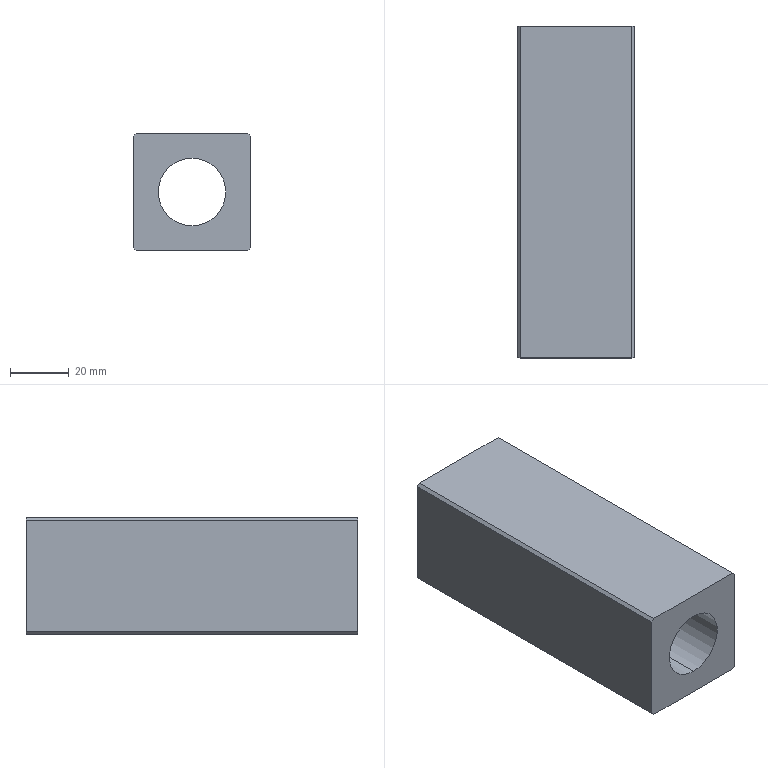Component | SolidWorks | BearingLiftingModule-1_CylinderLiftingModule-1_CDQ2B20-40DZ-L-M9B_0_0_0-1_CHEN123-AA-25-1 | 1 solid | 18 faces | box 40 x 113 x 40 mm | volume 118001 mm3 | plane 12 | cylinder 6 | commonest cylinder face diameters 30 x2 23 x2 28 x2
build123d program:
from build123d import *

# Parameters (mm, degrees)
SKETCH1_W           = 40
SKETCH1_H           = 40
BOSS_EXTRUDE1_DEPTH = 113
SKETCH2_R           = 11.5
CUT_EXTRUDE1_DEPTH  = 117.486
SKETCH3_R           = 14
CUT_EXTRUDE2_DEPTH  = 63
SKETCH4_R           = 15
CUT_EXTRUDE3_DEPTH  = 33
CHAMFER1_SIZE       = 1


with BuildPart() as part:
    # Sketch1 → Boss-Extrude1 (new body)
    with BuildSketch(Plane.XY):
        Rectangle(SKETCH1_W, SKETCH1_H)
    extrude(amount=BOSS_EXTRUDE1_DEPTH)

    # Sketch2 → Cut-Extrude1 (cut, through all)
    with BuildSketch(Plane.XY.offset(113)):
        Circle(SKETCH2_R)
    extrude(amount=-CUT_EXTRUDE1_DEPTH, mode=Mode.SUBTRACT)

    # Sketch3 → Cut-Extrude2 (cut)
    with BuildSketch(Plane(origin=(0, 0, 0), x_dir=(-1, 0, 0), z_dir=(0, 0, -1))):
        Circle(SKETCH3_R)
    extrude(amount=-CUT_EXTRUDE2_DEPTH, mode=Mode.SUBTRACT)

    # Sketch4 → Cut-Extrude3 (cut)
    with BuildSketch(Plane(origin=(0, 0, 0), x_dir=(-1, 0, 0), z_dir=(0, 0, -1))):
        Circle(SKETCH4_R)
    extrude(amount=-CUT_EXTRUDE3_DEPTH, mode=Mode.SUBTRACT)

    # Chamfer1
    chamfer1_edges = [part.edges().sort_by_distance(p)[0] for p in [
        (20, -20, 56.5),
        (-20, -20, 56.5),
        (-20, 20, 56.5),
        (20, 20, 56.5),
    ]]
    chamfer(chamfer1_edges, length=CHAMFER1_SIZE)


solid = part.part

# Placed as in the assembly
solid = solid.moved(Location((69.999, 21.801, 30), (90, 0, 0)))
STEP:
#1=CARTESIAN_POINT('',(2.756,-0.4409,1.772));
#2=VERTEX_POINT('',#1);
#3=CARTESIAN_POINT('',(2.756,-0.4409,0.5906));
#4=VERTEX_POINT('',#3);
#5=CARTESIAN_POINT('',(2.756,-0.4409,1.181));
#6=DIRECTION('',(0.,1.,-0.));
#7=DIRECTION('',(0.,0.,-1.));
#8=AXIS2_PLACEMENT_3D('',#5,#6,#7);
#9=CIRCLE('',#8,0.5906);
#10=EDGE_CURVE('',#2,#4,#9,.T.);
#11=ORIENTED_EDGE('',*,*,#10,.F.);
#12=CARTESIAN_POINT('',(2.756,0.8583,1.772));
#13=VERTEX_POINT('',#12);
#14=CARTESIAN_POINT('',(2.756,-0.4409,1.772));
#15=DIRECTION('',(0.,1.,-0.));
#16=VECTOR('',#15,39.37);
#17=LINE('',#14,#16);
#18=EDGE_CURVE('',#2,#13,#17,.T.);
#19=ORIENTED_EDGE('',*,*,#18,.T.);
#20=CARTESIAN_POINT('',(2.756,0.8583,0.5906));
#21=VERTEX_POINT('',#20);
#22=CARTESIAN_POINT('',(2.756,0.8583,1.181));
#23=DIRECTION('',(0.,1.,-0.));
#24=DIRECTION('',(0.,0.,-1.));
#25=AXIS2_PLACEMENT_3D('',#22,#23,#24);
#26=CIRCLE('',#25,0.5906);
#27=EDGE_CURVE('',#13,#21,#26,.T.);
#28=ORIENTED_EDGE('',*,*,#27,.T.);
#29=CARTESIAN_POINT('',(2.756,-0.4409,0.5906));
#30=DIRECTION('',(0.,1.,-0.));
#31=VECTOR('',#30,39.37);
#32=LINE('',#29,#31);
#33=EDGE_CURVE('',#4,#21,#32,.T.);
#34=ORIENTED_EDGE('',*,*,#33,.F.);
#35=EDGE_LOOP('',(#11,#19,#28,#34));
#36=FACE_OUTER_BOUND('',#35,.T.);
#37=CARTESIAN_POINT('',(2.756,-0.4409,1.181));
#38=DIRECTION('',(0.,1.,-0.));
#39=DIRECTION('',(0.,0.,-1.));
#40=AXIS2_PLACEMENT_3D('',#37,#38,#39);
#41=CYLINDRICAL_SURFACE('',#40,0.5906);
#42=ADVANCED_FACE('',(#36),#41,.F.);
#43=CARTESIAN_POINT('',(2.756,-1.622,0.7283));
#44=VERTEX_POINT('',#43);
#45=CARTESIAN_POINT('',(2.756,-1.622,1.634));
#46=VERTEX_POINT('',#45);
#47=CARTESIAN_POINT('',(2.756,-1.622,1.181));
#48=DIRECTION('',(0.,-1.,0.));
#49=DIRECTION('',(0.,0.,-1.));
#50=AXIS2_PLACEMENT_3D('',#47,#48,#49);
#51=CIRCLE('',#50,0.4528);
#52=EDGE_CURVE('',#44,#46,#51,.T.);
#53=ORIENTED_EDGE('',*,*,#52,.F.);
#54=CARTESIAN_POINT('',(2.756,-3.591,0.7283));
#55=VERTEX_POINT('',#54);
#56=CARTESIAN_POINT('',(2.756,0.8583,0.7283));
#57=DIRECTION('',(0.,-1.,0.));
#58=VECTOR('',#57,39.37);
#59=LINE('',#56,#58);
#60=EDGE_CURVE('',#44,#55,#59,.T.);
#61=ORIENTED_EDGE('',*,*,#60,.T.);
#62=CARTESIAN_POINT('',(2.756,-3.591,1.634));
#63=VERTEX_POINT('',#62);
#64=CARTESIAN_POINT('',(2.756,-3.591,1.181));
#65=DIRECTION('',(0.,-1.,0.));
#66=DIRECTION('',(0.,0.,1.));
#67=AXIS2_PLACEMENT_3D('',#64,#65,#66);
#68=CIRCLE('',#67,0.4528);
#69=EDGE_CURVE('',#55,#63,#68,.T.);
#70=ORIENTED_EDGE('',*,*,#69,.T.);
#71=CARTESIAN_POINT('',(2.756,0.8583,1.634));
#72=DIRECTION('',(0.,-1.,0.));
#73=VECTOR('',#72,39.37);
#74=LINE('',#71,#73);
#75=EDGE_CURVE('',#46,#63,#74,.T.);
#76=ORIENTED_EDGE('',*,*,#75,.F.);
#77=EDGE_LOOP('',(#53,#61,#70,#76));
#78=FACE_OUTER_BOUND('',#77,.T.);
#79=CARTESIAN_POINT('',(2.756,0.8583,1.181));
#80=DIRECTION('',(0.,-1.,0.));
#81=DIRECTION('',(0.,0.,1.));
#82=AXIS2_PLACEMENT_3D('',#79,#80,#81);
#83=CYLINDRICAL_SURFACE('',#82,0.4528);
#84=ADVANCED_FACE('',(#78),#83,.F.);
#85=CARTESIAN_POINT('',(2.756,-1.622,1.732));
#86=VERTEX_POINT('',#85);
#87=CARTESIAN_POINT('',(2.756,-1.622,0.6299));
#88=VERTEX_POINT('',#87);
#89=CARTESIAN_POINT('',(2.756,-1.622,1.181));
#90=DIRECTION('',(0.,1.,-0.));
#91=DIRECTION('',(0.,0.,-1.));
#92=AXIS2_PLACEMENT_3D('',#89,#90,#91);
#93=CIRCLE('',#92,0.5512);
#94=EDGE_CURVE('',#86,#88,#93,.T.);
#95=ORIENTED_EDGE('',*,*,#94,.F.);
#96=CARTESIAN_POINT('',(2.756,-0.4409,1.732));
#97=VERTEX_POINT('',#96);
#98=CARTESIAN_POINT('',(2.756,-1.622,1.732));
#99=DIRECTION('',(0.,1.,-0.));
#100=VECTOR('',#99,39.37);
#101=LINE('',#98,#100);
#102=EDGE_CURVE('',#86,#97,#101,.T.);
#103=ORIENTED_EDGE('',*,*,#102,.T.);
#104=CARTESIAN_POINT('',(2.756,-0.4409,0.6299));
#105=VERTEX_POINT('',#104);
#106=CARTESIAN_POINT('',(2.756,-0.4409,1.181));
#107=DIRECTION('',(0.,-1.,0.));
#108=DIRECTION('',(0.,0.,-1.));
#109=AXIS2_PLACEMENT_3D('',#106,#107,#108);
#110=CIRCLE('',#109,0.5512);
#111=EDGE_CURVE('',#105,#97,#110,.T.);
#112=ORIENTED_EDGE('',*,*,#111,.F.);
#113=CARTESIAN_POINT('',(2.756,-1.622,0.6299));
#114=DIRECTION('',(0.,1.,-0.));
#115=VECTOR('',#114,39.37);
#116=LINE('',#113,#115);
#117=EDGE_CURVE('',#88,#105,#116,.T.);
#118=ORIENTED_EDGE('',*,*,#117,.F.);
#119=EDGE_LOOP('',(#95,#103,#112,#118));
#120=FACE_OUTER_BOUND('',#119,.T.);
#121=CARTESIAN_POINT('',(2.756,-1.622,1.181));
#122=DIRECTION('',(0.,1.,-0.));
#123=DIRECTION('',(0.,0.,-1.));
#124=AXIS2_PLACEMENT_3D('',#121,#122,#123);
#125=CYLINDRICAL_SURFACE('',#124,0.5512);
#126=ADVANCED_FACE('',(#120),#125,.F.);
#127=ORIENTED_EDGE('',*,*,#102,.F.);
#128=CARTESIAN_POINT('',(2.756,-1.622,1.181));
#129=DIRECTION('',(0.,1.,-0.));
#130=DIRECTION('',(0.,0.,-1.));
#131=AXIS2_PLACEMENT_3D('',#128,#129,#130);
#132=CIRCLE('',#131,0.5512);
#133=EDGE_CURVE('',#88,#86,#132,.T.);
#134=ORIENTED_EDGE('',*,*,#133,.F.);
#135=ORIENTED_EDGE('',*,*,#117,.T.);
#136=CARTESIAN_POINT('',(2.756,-0.4409,1.181));
#137=DIRECTION('',(0.,-1.,0.));
#138=DIRECTION('',(0.,0.,-1.));
#139=AXIS2_PLACEMENT_3D('',#136,#137,#138);
#140=CIRCLE('',#139,0.5512);
#141=EDGE_CURVE('',#97,#105,#140,.T.);
#142=ORIENTED_EDGE('',*,*,#141,.F.);
#143=EDGE_LOOP('',(#127,#134,#135,#142));
#144=FACE_OUTER_BOUND('',#143,.T.);
#145=CARTESIAN_POINT('',(2.756,-1.622,1.181));
#146=DIRECTION('',(0.,1.,-0.));
#147=DIRECTION('',(0.,0.,-1.));
#148=AXIS2_PLACEMENT_3D('',#145,#146,#147);
#149=CYLINDRICAL_SURFACE('',#148,0.5512);
#150=ADVANCED_FACE('',(#144),#149,.F.);
#151=ORIENTED_EDGE('',*,*,#60,.F.);
#152=CARTESIAN_POINT('',(2.756,-1.622,1.181));
#153=DIRECTION('',(0.,-1.,0.));
#154=DIRECTION('',(0.,0.,-1.));
#155=AXIS2_PLACEMENT_3D('',#152,#153,#154);
#156=CIRCLE('',#155,0.4528);
#157=EDGE_CURVE('',#46,#44,#156,.T.);
#158=ORIENTED_EDGE('',*,*,#157,.F.);
#159=ORIENTED_EDGE('',*,*,#75,.T.);
#160=CARTESIAN_POINT('',(2.756,-3.591,1.181));
#161=DIRECTION('',(0.,-1.,0.));
#162=DIRECTION('',(0.,0.,1.));
#163=AXIS2_PLACEMENT_3D('',#160,#161,#162);
#164=CIRCLE('',#163,0.4528);
#165=EDGE_CURVE('',#63,#55,#164,.T.);
#166=ORIENTED_EDGE('',*,*,#165,.T.);
#167=EDGE_LOOP('',(#151,#158,#159,#166));
#168=FACE_OUTER_BOUND('',#167,.T.);
#169=CARTESIAN_POINT('',(2.756,0.8583,1.181));
#170=DIRECTION('',(0.,-1.,0.));
#171=DIRECTION('',(0.,0.,1.));
#172=AXIS2_PLACEMENT_3D('',#169,#170,#171);
#173=CYLINDRICAL_SURFACE('',#172,0.4528);
#174=ADVANCED_FACE('',(#168),#173,.F.);
#175=CARTESIAN_POINT('',(3.504,0.8583,1.969));
#176=VERTEX_POINT('',#175);
#177=CARTESIAN_POINT('',(2.008,0.8583,1.969));
#178=VERTEX_POINT('',#177);
#179=CARTESIAN_POINT('',(3.543,0.8583,1.969));
#180=DIRECTION('',(-1.,0.,0.));
#181=VECTOR('',#180,39.37);
#182=LINE('',#179,#181);
#183=EDGE_CURVE('',#176,#178,#182,.T.);
#184=ORIENTED_EDGE('',*,*,#183,.T.);
#185=CARTESIAN_POINT('',(2.008,-3.591,1.969));
#186=VERTEX_POINT('',#185);
#187=CARTESIAN_POINT('',(2.008,-3.591,1.969));
#188=DIRECTION('',(0.,-1.,0.));
#189=VECTOR('',#188,39.37);
#190=LINE('',#187,#189);
#191=EDGE_CURVE('',#178,#186,#190,.T.);
#192=ORIENTED_EDGE('',*,*,#191,.T.);
#193=CARTESIAN_POINT('',(3.504,-3.591,1.969));
#194=VERTEX_POINT('',#193);
#195=CARTESIAN_POINT('',(3.543,-3.591,1.969));
#196=DIRECTION('',(-1.,0.,0.));
#197=VECTOR('',#196,39.37);
#198=LINE('',#195,#197);
#199=EDGE_CURVE('',#194,#186,#198,.T.);
#200=ORIENTED_EDGE('',*,*,#199,.F.);
#201=CARTESIAN_POINT('',(3.504,-3.591,1.969));
#202=DIRECTION('',(0.,1.,-0.));
#203=VECTOR('',#202,39.37);
#204=LINE('',#201,#203);
#205=EDGE_CURVE('',#194,#176,#204,.T.);
#206=ORIENTED_EDGE('',*,*,#205,.T.);
#207=EDGE_LOOP('',(#184,#192,#200,#206));
#208=FACE_OUTER_BOUND('',#207,.T.);
#209=CARTESIAN_POINT('',(3.543,-3.591,1.969));
#210=DIRECTION('',(-0.,-0.,-1.));
#211=DIRECTION('',(0.,-1.,0.));
#212=AXIS2_PLACEMENT_3D('',#209,#210,#211);
#213=PLANE('',#212);
#214=ADVANCED_FACE('',(#208),#213,.F.);
#215=CARTESIAN_POINT('',(1.968,0.8583,1.929));
#216=VERTEX_POINT('',#215);
#217=CARTESIAN_POINT('',(1.968,0.8583,0.4331));
#218=VERTEX_POINT('',#217);
#219=CARTESIAN_POINT('',(1.968,0.8583,0.3937));
#220=DIRECTION('',(-0.,-0.,-1.));
#221=VECTOR('',#220,39.37);
#222=LINE('',#219,#221);
#223=EDGE_CURVE('',#216,#218,#222,.T.);
#224=ORIENTED_EDGE('',*,*,#223,.T.);
#225=CARTESIAN_POINT('',(1.968,-3.591,0.4331));
#226=VERTEX_POINT('',#225);
#227=CARTESIAN_POINT('',(1.968,-3.591,0.4331));
#228=DIRECTION('',(0.,-1.,0.));
#229=VECTOR('',#228,39.37);
#230=LINE('',#227,#229);
#231=EDGE_CURVE('',#218,#226,#230,.T.);
#232=ORIENTED_EDGE('',*,*,#231,.T.);
#233=CARTESIAN_POINT('',(1.968,-3.591,1.929));
#234=VERTEX_POINT('',#233);
#235=CARTESIAN_POINT('',(1.968,-3.591,0.3937));
#236=DIRECTION('',(-0.,-0.,-1.));
#237=VECTOR('',#236,39.37);
#238=LINE('',#235,#237);
#239=EDGE_CURVE('',#234,#226,#238,.T.);
#240=ORIENTED_EDGE('',*,*,#239,.F.);
#241=CARTESIAN_POINT('',(1.968,-3.591,1.929));
#242=DIRECTION('',(0.,1.,-0.));
#243=VECTOR('',#242,39.37);
#244=LINE('',#241,#243);
#245=EDGE_CURVE('',#234,#216,#244,.T.);
#246=ORIENTED_EDGE('',*,*,#245,.T.);
#247=EDGE_LOOP('',(#224,#232,#240,#246));
#248=FACE_OUTER_BOUND('',#247,.T.);
#249=CARTESIAN_POINT('',(1.968,-3.591,0.3937));
#250=DIRECTION('',(1.,-0.,-0.));
#251=DIRECTION('',(0.,1.,-0.));
#252=AXIS2_PLACEMENT_3D('',#249,#250,#251);
#253=PLANE('',#252);
#254=ADVANCED_FACE('',(#248),#253,.F.);
#255=CARTESIAN_POINT('',(2.008,0.8583,0.3937));
#256=VERTEX_POINT('',#255);
#257=CARTESIAN_POINT('',(3.504,0.8583,0.3937));
#258=VERTEX_POINT('',#257);
#259=CARTESIAN_POINT('',(3.543,0.8583,0.3937));
#260=DIRECTION('',(1.,0.,-0.));
#261=VECTOR('',#260,39.37);
#262=LINE('',#259,#261);
#263=EDGE_CURVE('',#256,#258,#262,.T.);
#264=ORIENTED_EDGE('',*,*,#263,.T.);
#265=CARTESIAN_POINT('',(3.504,-3.591,0.3937));
#266=VERTEX_POINT('',#265);
#267=CARTESIAN_POINT('',(3.504,-3.591,0.3937));
#268=DIRECTION('',(0.,-1.,0.));
#269=VECTOR('',#268,39.37);
#270=LINE('',#267,#269);
#271=EDGE_CURVE('',#258,#266,#270,.T.);
#272=ORIENTED_EDGE('',*,*,#271,.T.);
#273=CARTESIAN_POINT('',(2.008,-3.591,0.3937));
#274=VERTEX_POINT('',#273);
#275=CARTESIAN_POINT('',(3.543,-3.591,0.3937));
#276=DIRECTION('',(1.,0.,-0.));
#277=VECTOR('',#276,39.37);
#278=LINE('',#275,#277);
#279=EDGE_CURVE('',#274,#266,#278,.T.);
#280=ORIENTED_EDGE('',*,*,#279,.F.);
#281=CARTESIAN_POINT('',(2.008,-3.591,0.3937));
#282=DIRECTION('',(0.,1.,-0.));
#283=VECTOR('',#282,39.37);
#284=LINE('',#281,#283);
#285=EDGE_CURVE('',#274,#256,#284,.T.);
#286=ORIENTED_EDGE('',*,*,#285,.T.);
#287=EDGE_LOOP('',(#264,#272,#280,#286));
#288=FACE_OUTER_BOUND('',#287,.T.);
#289=CARTESIAN_POINT('',(3.543,-3.591,0.3937));
#290=DIRECTION('',(0.,0.,1.));
#291=DIRECTION('',(0.,1.,-0.));
#292=AXIS2_PLACEMENT_3D('',#289,#290,#291);
#293=PLANE('',#292);
#294=ADVANCED_FACE('',(#288),#293,.F.);
#295=CARTESIAN_POINT('',(3.543,-3.591,0.4331));
#296=VERTEX_POINT('',#295);
#297=CARTESIAN_POINT('',(3.543,-3.591,1.929));
#298=VERTEX_POINT('',#297);
#299=CARTESIAN_POINT('',(3.543,-3.591,0.3937));
#300=DIRECTION('',(0.,0.,1.));
#301=VECTOR('',#300,39.37);
#302=LINE('',#299,#301);
#303=EDGE_CURVE('',#296,#298,#302,.T.);
#304=ORIENTED_EDGE('',*,*,#303,.F.);
#305=CARTESIAN_POINT('',(3.543,0.8583,0.4331));
#306=VERTEX_POINT('',#305);
#307=CARTESIAN_POINT('',(3.543,-3.591,0.4331));
#308=DIRECTION('',(0.,1.,-0.));
#309=VECTOR('',#308,39.37);
#310=LINE('',#307,#309);
#311=EDGE_CURVE('',#296,#306,#310,.T.);
#312=ORIENTED_EDGE('',*,*,#311,.T.);
#313=CARTESIAN_POINT('',(3.543,0.8583,1.929));
#314=VERTEX_POINT('',#313);
#315=CARTESIAN_POINT('',(3.543,0.8583,0.3937));
#316=DIRECTION('',(0.,0.,1.));
#317=VECTOR('',#316,39.37);
#318=LINE('',#315,#317);
#319=EDGE_CURVE('',#306,#314,#318,.T.);
#320=ORIENTED_EDGE('',*,*,#319,.T.);
#321=CARTESIAN_POINT('',(3.543,-3.591,1.929));
#322=DIRECTION('',(0.,-1.,0.));
#323=VECTOR('',#322,39.37);
#324=LINE('',#321,#323);
#325=EDGE_CURVE('',#314,#298,#324,.T.);
#326=ORIENTED_EDGE('',*,*,#325,.T.);
#327=EDGE_LOOP('',(#304,#312,#320,#326));
#328=FACE_OUTER_BOUND('',#327,.T.);
#329=CARTESIAN_POINT('',(3.543,-3.591,0.3937));
#330=DIRECTION('',(-1.,0.,0.));
#331=DIRECTION('',(0.,-1.,0.));
#332=AXIS2_PLACEMENT_3D('',#329,#330,#331);
#333=PLANE('',#332);
#334=ADVANCED_FACE('',(#328),#333,.F.);
#335=ORIENTED_EDGE('',*,*,#165,.F.);
#336=ORIENTED_EDGE('',*,*,#69,.F.);
#337=EDGE_LOOP('',(#335,#336));
#338=FACE_BOUND('',#337,.T.);
#339=ORIENTED_EDGE('',*,*,#279,.T.);
#340=CARTESIAN_POINT('',(3.543,-3.591,0.4331));
#341=DIRECTION('',(0.7071,0.,0.7071));
#342=VECTOR('',#341,39.37);
#343=LINE('',#340,#342);
#344=EDGE_CURVE('',#266,#296,#343,.T.);
#345=ORIENTED_EDGE('',*,*,#344,.T.);
#346=ORIENTED_EDGE('',*,*,#303,.T.);
#347=CARTESIAN_POINT('',(3.504,-3.591,1.969));
#348=DIRECTION('',(-0.7071,0.,0.7071));
#349=VECTOR('',#348,39.37);
#350=LINE('',#347,#349);
#351=EDGE_CURVE('',#298,#194,#350,.T.);
#352=ORIENTED_EDGE('',*,*,#351,.T.);
#353=ORIENTED_EDGE('',*,*,#199,.T.);
#354=CARTESIAN_POINT('',(1.968,-3.591,1.929));
#355=DIRECTION('',(-0.7071,-0.,-0.7071));
#356=VECTOR('',#355,39.37);
#357=LINE('',#354,#356);
#358=EDGE_CURVE('',#186,#234,#357,.T.);
#359=ORIENTED_EDGE('',*,*,#358,.T.);
#360=ORIENTED_EDGE('',*,*,#239,.T.);
#361=CARTESIAN_POINT('',(2.008,-3.591,0.3937));
#362=DIRECTION('',(0.7071,-0.,-0.7071));
#363=VECTOR('',#362,39.37);
#364=LINE('',#361,#363);
#365=EDGE_CURVE('',#226,#274,#364,.T.);
#366=ORIENTED_EDGE('',*,*,#365,.T.);
#367=EDGE_LOOP('',(#339,#345,#346,#352,#353,#359,#360,#366));
#368=FACE_OUTER_BOUND('',#367,.T.);
#369=CARTESIAN_POINT('',(2.756,-3.591,1.181));
#370=DIRECTION('',(0.,1.,-0.));
#371=DIRECTION('',(-0.,-0.,-1.));
#372=AXIS2_PLACEMENT_3D('',#369,#370,#371);
#373=PLANE('',#372);
#374=ADVANCED_FACE('',(#338,#368),#373,.F.);
#375=CARTESIAN_POINT('',(2.756,0.8583,1.181));
#376=DIRECTION('',(0.,1.,-0.));
#377=DIRECTION('',(0.,0.,-1.));
#378=AXIS2_PLACEMENT_3D('',#375,#376,#377);
#379=CIRCLE('',#378,0.5906);
#380=EDGE_CURVE('',#21,#13,#379,.T.);
#381=ORIENTED_EDGE('',*,*,#380,.F.);
#382=ORIENTED_EDGE('',*,*,#27,.F.);
#383=EDGE_LOOP('',(#381,#382));
#384=FACE_BOUND('',#383,.T.);
#385=ORIENTED_EDGE('',*,*,#319,.F.);
#386=CARTESIAN_POINT('',(3.524,0.8583,0.4134));
#387=DIRECTION('',(-0.7071,-0.,-0.7071));
#388=VECTOR('',#387,39.37);
#389=LINE('',#386,#388);
#390=EDGE_CURVE('',#306,#258,#389,.T.);
#391=ORIENTED_EDGE('',*,*,#390,.T.);
#392=ORIENTED_EDGE('',*,*,#263,.F.);
#393=CARTESIAN_POINT('',(1.988,0.8583,0.4134));
#394=DIRECTION('',(-0.7071,0.,0.7071));
#395=VECTOR('',#394,39.37);
#396=LINE('',#393,#395);
#397=EDGE_CURVE('',#256,#218,#396,.T.);
#398=ORIENTED_EDGE('',*,*,#397,.T.);
#399=ORIENTED_EDGE('',*,*,#223,.F.);
#400=CARTESIAN_POINT('',(1.988,0.8583,1.949));
#401=DIRECTION('',(0.7071,0.,0.7071));
#402=VECTOR('',#401,39.37);
#403=LINE('',#400,#402);
#404=EDGE_CURVE('',#216,#178,#403,.T.);
#405=ORIENTED_EDGE('',*,*,#404,.T.);
#406=ORIENTED_EDGE('',*,*,#183,.F.);
#407=CARTESIAN_POINT('',(3.524,0.8583,1.949));
#408=DIRECTION('',(0.7071,-0.,-0.7071));
#409=VECTOR('',#408,39.37);
#410=LINE('',#407,#409);
#411=EDGE_CURVE('',#176,#314,#410,.T.);
#412=ORIENTED_EDGE('',*,*,#411,.T.);
#413=EDGE_LOOP('',(#385,#391,#392,#398,#399,#405,#406,#412));
#414=FACE_OUTER_BOUND('',#413,.T.);
#415=CARTESIAN_POINT('',(2.756,0.8583,1.181));
#416=DIRECTION('',(0.,1.,-0.));
#417=DIRECTION('',(-0.,-0.,-1.));
#418=AXIS2_PLACEMENT_3D('',#415,#416,#417);
#419=PLANE('',#418);
#420=ADVANCED_FACE('',(#384,#414),#419,.T.);
#421=ORIENTED_EDGE('',*,*,#133,.T.);
#422=ORIENTED_EDGE('',*,*,#94,.T.);
#423=EDGE_LOOP('',(#421,#422));
#424=FACE_OUTER_BOUND('',#423,.T.);
#425=ORIENTED_EDGE('',*,*,#157,.T.);
#426=ORIENTED_EDGE('',*,*,#52,.T.);
#427=EDGE_LOOP('',(#425,#426));
#428=FACE_BOUND('',#427,.T.);
#429=CARTESIAN_POINT('',(2.756,-1.622,1.181));
#430=DIRECTION('',(0.,1.,-0.));
#431=DIRECTION('',(-0.,-0.,-1.));
#432=AXIS2_PLACEMENT_3D('',#429,#430,#431);
#433=PLANE('',#432);
#434=ADVANCED_FACE('',(#424,#428),#433,.T.);
#435=CARTESIAN_POINT('',(2.756,-0.4409,1.181));
#436=DIRECTION('',(0.,1.,-0.));
#437=DIRECTION('',(0.,0.,-1.));
#438=AXIS2_PLACEMENT_3D('',#435,#436,#437);
#439=CIRCLE('',#438,0.5906);
#440=EDGE_CURVE('',#4,#2,#439,.T.);
#441=ORIENTED_EDGE('',*,*,#440,.T.);
#442=ORIENTED_EDGE('',*,*,#10,.T.);
#443=EDGE_LOOP('',(#441,#442));
#444=FACE_OUTER_BOUND('',#443,.T.);
#445=ORIENTED_EDGE('',*,*,#111,.T.);
#446=ORIENTED_EDGE('',*,*,#141,.T.);
#447=EDGE_LOOP('',(#445,#446));
#448=FACE_BOUND('',#447,.T.);
#449=CARTESIAN_POINT('',(2.756,-0.4409,1.181));
#450=DIRECTION('',(0.,1.,-0.));
#451=DIRECTION('',(-0.,-0.,-1.));
#452=AXIS2_PLACEMENT_3D('',#449,#450,#451);
#453=PLANE('',#452);
#454=ADVANCED_FACE('',(#444,#448),#453,.T.);
#455=ORIENTED_EDGE('',*,*,#18,.F.);
#456=ORIENTED_EDGE('',*,*,#440,.F.);
#457=ORIENTED_EDGE('',*,*,#33,.T.);
#458=ORIENTED_EDGE('',*,*,#380,.T.);
#459=EDGE_LOOP('',(#455,#456,#457,#458));
#460=FACE_OUTER_BOUND('',#459,.T.);
#461=CARTESIAN_POINT('',(2.756,-0.4409,1.181));
#462=DIRECTION('',(0.,1.,-0.));
#463=DIRECTION('',(0.,0.,-1.));
#464=AXIS2_PLACEMENT_3D('',#461,#462,#463);
#465=CYLINDRICAL_SURFACE('',#464,0.5906);
#466=ADVANCED_FACE('',(#460),#465,.F.);
#467=ORIENTED_EDGE('',*,*,#344,.F.);
#468=ORIENTED_EDGE('',*,*,#271,.F.);
#469=ORIENTED_EDGE('',*,*,#390,.F.);
#470=ORIENTED_EDGE('',*,*,#311,.F.);
#471=EDGE_LOOP('',(#467,#468,#469,#470));
#472=FACE_OUTER_BOUND('',#471,.T.);
#473=CARTESIAN_POINT('',(3.543,-3.591,0.4331));
#474=DIRECTION('',(-0.7071,0.,0.7071));
#475=DIRECTION('',(0.,1.,-0.));
#476=AXIS2_PLACEMENT_3D('',#473,#474,#475);
#477=PLANE('',#476);
#478=ADVANCED_FACE('',(#472),#477,.F.);
#479=ORIENTED_EDGE('',*,*,#365,.F.);
#480=ORIENTED_EDGE('',*,*,#231,.F.);
#481=ORIENTED_EDGE('',*,*,#397,.F.);
#482=ORIENTED_EDGE('',*,*,#285,.F.);
#483=EDGE_LOOP('',(#479,#480,#481,#482));
#484=FACE_OUTER_BOUND('',#483,.T.);
#485=CARTESIAN_POINT('',(2.008,-3.591,0.3937));
#486=DIRECTION('',(0.7071,0.,0.7071));
#487=DIRECTION('',(0.,1.,-0.));
#488=AXIS2_PLACEMENT_3D('',#485,#486,#487);
#489=PLANE('',#488);
#490=ADVANCED_FACE('',(#484),#489,.F.);
#491=ORIENTED_EDGE('',*,*,#358,.F.);
#492=ORIENTED_EDGE('',*,*,#191,.F.);
#493=ORIENTED_EDGE('',*,*,#404,.F.);
#494=ORIENTED_EDGE('',*,*,#245,.F.);
#495=EDGE_LOOP('',(#491,#492,#493,#494));
#496=FACE_OUTER_BOUND('',#495,.T.);
#497=CARTESIAN_POINT('',(1.968,-3.591,1.929));
#498=DIRECTION('',(0.7071,-0.,-0.7071));
#499=DIRECTION('',(0.,1.,-0.));
#500=AXIS2_PLACEMENT_3D('',#497,#498,#499);
#501=PLANE('',#500);
#502=ADVANCED_FACE('',(#496),#501,.F.);
#503=ORIENTED_EDGE('',*,*,#351,.F.);
#504=ORIENTED_EDGE('',*,*,#325,.F.);
#505=ORIENTED_EDGE('',*,*,#411,.F.);
#506=ORIENTED_EDGE('',*,*,#205,.F.);
#507=EDGE_LOOP('',(#503,#504,#505,#506));
#508=FACE_OUTER_BOUND('',#507,.T.);
#509=CARTESIAN_POINT('',(3.504,-3.591,1.969));
#510=DIRECTION('',(-0.7071,-0.,-0.7071));
#511=DIRECTION('',(0.,1.,-0.));
#512=AXIS2_PLACEMENT_3D('',#509,#510,#511);
#513=PLANE('',#512);
#514=ADVANCED_FACE('',(#508),#513,.F.);
#515=CLOSED_SHELL('',(#42,#84,#126,#150,#174,#214,#254,#294,#334,#374,#420,#434,#454,#466,#478,#490,#502,#514));
#516=MANIFOLD_SOLID_BREP('',#515);
#517=CARTESIAN_POINT('',(0.,0.,0.));
#518=DIRECTION('',(0.,0.,1.));
#519=DIRECTION('',(1.,0.,0.));
#520=AXIS2_PLACEMENT_3D('',#517,#518,#519);
#521=(LENGTH_UNIT()NAMED_UNIT(*)SI_UNIT($,.METRE.));
#522=LENGTH_MEASURE_WITH_UNIT(LENGTH_MEASURE(0.0254),#521);
#523=DIMENSIONAL_EXPONENTS(1.,0.,0.,0.,0.,0.,0.);
#524=(CONVERSION_BASED_UNIT('',#522)LENGTH_UNIT()NAMED_UNIT(#523));
#525=UNCERTAINTY_MEASURE_WITH_UNIT(LENGTH_MEASURE(0.00001),#524,'','');
#526=(NAMED_UNIT(*)PLANE_ANGLE_UNIT()SI_UNIT($,.RADIAN.));
#527=(NAMED_UNIT(*)SI_UNIT($,.STERADIAN.)SOLID_ANGLE_UNIT());
#528=(GEOMETRIC_REPRESENTATION_CONTEXT(3)GLOBAL_UNCERTAINTY_ASSIGNED_CONTEXT((#525))GLOBAL_UNIT_ASSIGNED_CONTEXT((#524,#526,#527))REPRESENTATION_CONTEXT('',''));
#529=ADVANCED_BREP_SHAPE_REPRESENTATION('',(#516,#520),#528);
#530=COLOUR_RGB('',0.7922,0.8196,0.9333);
#531=FILL_AREA_STYLE_COLOUR('',#530);
#532=FILL_AREA_STYLE('',(#531));
#533=SURFACE_STYLE_FILL_AREA(#532);
#534=SURFACE_SIDE_STYLE('',(#533));
#535=SURFACE_STYLE_USAGE(.BOTH.,#534);
#536=PRESENTATION_STYLE_ASSIGNMENT((#535));
#537=STYLED_ITEM('',(#536),#516);
#538=PRESENTATION_LAYER_ASSIGNMENT('','',(#537));
#539=(LENGTH_UNIT()NAMED_UNIT(*)SI_UNIT($,.METRE.));
#540=LENGTH_MEASURE_WITH_UNIT(LENGTH_MEASURE(0.0254),#539);
#541=DIMENSIONAL_EXPONENTS(1.,0.,0.,0.,0.,0.,0.);
#542=(CONVERSION_BASED_UNIT('',#540)LENGTH_UNIT()NAMED_UNIT(#541));
#543=UNCERTAINTY_MEASURE_WITH_UNIT(LENGTH_MEASURE(0.00001),#542,'','');
#544=(NAMED_UNIT(*)PLANE_ANGLE_UNIT()SI_UNIT($,.RADIAN.));
#545=(NAMED_UNIT(*)SI_UNIT($,.STERADIAN.)SOLID_ANGLE_UNIT());
#546=(GEOMETRIC_REPRESENTATION_CONTEXT(3)GLOBAL_UNCERTAINTY_ASSIGNED_CONTEXT((#543))GLOBAL_UNIT_ASSIGNED_CONTEXT((#542,#544,#545))REPRESENTATION_CONTEXT('',''));
#547=MECHANICAL_DESIGN_GEOMETRIC_PRESENTATION_REPRESENTATION('',(#537),#546);